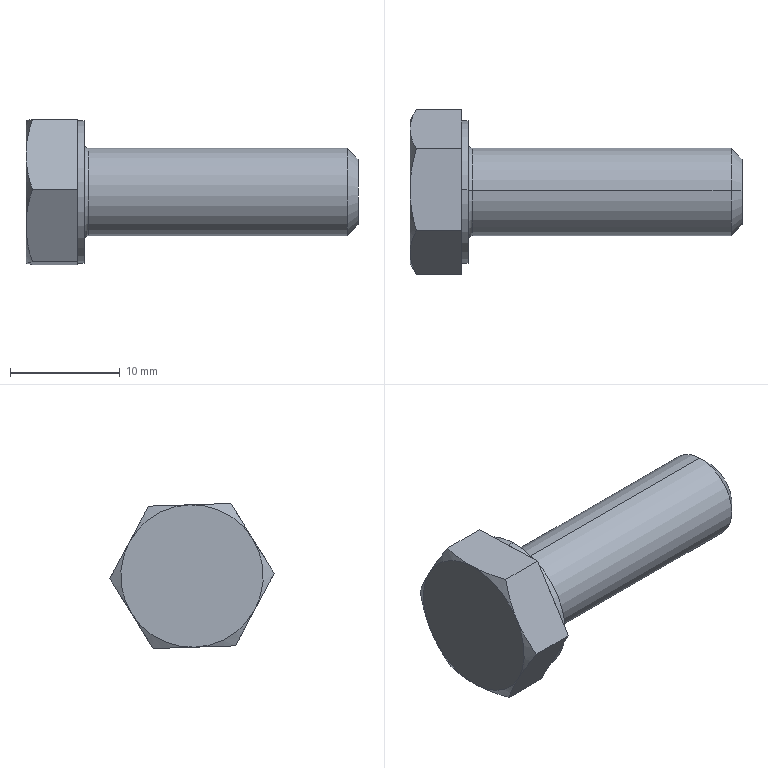Component | SolidWorks | GB_T5781-2000HexHeadBoltFullThreadC-gradeM8_25-1 | 1 solid | 29 faces | box 30.3 x 15 x 13.24 mm | volume 2011 mm3 | plane 15 | cone 8 | cylinder 4 | torus 2 | commonest cylinder face diameters 8 x2 13 x2
STEP:
#1=CARTESIAN_POINT('',(-21.77,0.005166,0.1574));
#2=VERTEX_POINT('',#1);
#3=CARTESIAN_POINT('',(-21.77,-0.005166,-0.1574));
#4=VERTEX_POINT('',#3);
#5=CARTESIAN_POINT('',(-21.77,0.,0.));
#6=DIRECTION('',(1.,0.,0.));
#7=DIRECTION('',(0.,-0.03281,-0.9995));
#8=AXIS2_PLACEMENT_3D('',#5,#6,#7);
#9=CIRCLE('',#8,0.1575);
#10=EDGE_CURVE('',#2,#4,#9,.T.);
#11=ORIENTED_EDGE('',*,*,#10,.F.);
#12=CARTESIAN_POINT('',(-21.786,0.005683,0.1731));
#13=VERTEX_POINT('',#12);
#14=CARTESIAN_POINT('',(-21.77,0.005683,0.1731));
#15=DIRECTION('',(0.,0.9995,-0.03281));
#16=DIRECTION('',(0.,0.03281,0.9995));
#17=AXIS2_PLACEMENT_3D('',#14,#15,#16);
#18=CIRCLE('',#17,0.01575);
#19=EDGE_CURVE('',#2,#13,#18,.T.);
#20=ORIENTED_EDGE('',*,*,#19,.T.);
#21=CARTESIAN_POINT('',(-21.786,-0.005683,-0.1731));
#22=VERTEX_POINT('',#21);
#23=CARTESIAN_POINT('',(-21.786,0.,0.));
#24=DIRECTION('',(-1.,0.,0.));
#25=DIRECTION('',(0.,-0.03281,-0.9995));
#26=AXIS2_PLACEMENT_3D('',#23,#24,#25);
#27=CIRCLE('',#26,0.1732);
#28=EDGE_CURVE('',#22,#13,#27,.T.);
#29=ORIENTED_EDGE('',*,*,#28,.F.);
#30=CARTESIAN_POINT('',(-21.77,-0.005683,-0.1731));
#31=DIRECTION('',(0.,-0.9995,0.03281));
#32=DIRECTION('',(0.,-0.03281,-0.9995));
#33=AXIS2_PLACEMENT_3D('',#30,#31,#32);
#34=CIRCLE('',#33,0.01575);
#35=EDGE_CURVE('',#4,#22,#34,.T.);
#36=ORIENTED_EDGE('',*,*,#35,.F.);
#37=EDGE_LOOP('',(#11,#20,#29,#36));
#38=FACE_OUTER_BOUND('',#37,.T.);
#39=CARTESIAN_POINT('',(-21.77,0.,0.));
#40=DIRECTION('',(1.,0.,0.));
#41=DIRECTION('',(0.,-0.03281,-0.9995));
#42=AXIS2_PLACEMENT_3D('',#39,#40,#41);
#43=TOROIDAL_SURFACE('',#42,0.1732,0.01575);
#44=ADVANCED_FACE('',(#38),#43,.F.);
#45=CARTESIAN_POINT('',(-20.802,-0.003875,-0.118));
#46=VERTEX_POINT('',#45);
#47=CARTESIAN_POINT('',(-20.802,0.003875,0.118));
#48=VERTEX_POINT('',#47);
#49=CARTESIAN_POINT('',(-20.802,0.,0.));
#50=DIRECTION('',(1.,0.,0.));
#51=DIRECTION('',(0.,0.03281,0.9995));
#52=AXIS2_PLACEMENT_3D('',#49,#50,#51);
#53=CIRCLE('',#52,0.1181);
#54=EDGE_CURVE('',#46,#48,#53,.T.);
#55=ORIENTED_EDGE('',*,*,#54,.F.);
#56=CARTESIAN_POINT('',(-20.841,-0.005166,-0.1574));
#57=VERTEX_POINT('',#56);
#58=CARTESIAN_POINT('',(-20.841,-0.005166,-0.1574));
#59=DIRECTION('',(-0.7071,-0.0232,-0.7067));
#60=VECTOR('',#59,39.37);
#61=LINE('',#58,#60);
#62=EDGE_CURVE('',#46,#57,#61,.T.);
#63=ORIENTED_EDGE('',*,*,#62,.T.);
#64=CARTESIAN_POINT('',(-20.841,0.005166,0.1574));
#65=VERTEX_POINT('',#64);
#66=CARTESIAN_POINT('',(-20.841,0.,0.));
#67=DIRECTION('',(-1.,0.,0.));
#68=DIRECTION('',(0.,0.03281,0.9995));
#69=AXIS2_PLACEMENT_3D('',#66,#67,#68);
#70=CIRCLE('',#69,0.1575);
#71=EDGE_CURVE('',#65,#57,#70,.T.);
#72=ORIENTED_EDGE('',*,*,#71,.F.);
#73=CARTESIAN_POINT('',(-20.841,0.005166,0.1574));
#74=DIRECTION('',(-0.7071,0.0232,0.7067));
#75=VECTOR('',#74,39.37);
#76=LINE('',#73,#75);
#77=EDGE_CURVE('',#48,#65,#76,.T.);
#78=ORIENTED_EDGE('',*,*,#77,.F.);
#79=EDGE_LOOP('',(#55,#63,#72,#78));
#80=FACE_OUTER_BOUND('',#79,.T.);
#81=CARTESIAN_POINT('',(-20.841,0.,0.));
#82=DIRECTION('',(-1.,0.,0.));
#83=DIRECTION('',(0.,0.03281,0.9995));
#84=AXIS2_PLACEMENT_3D('',#81,#82,#83);
#85=CONICAL_SURFACE('',#84,0.1575,0.7854);
#86=ADVANCED_FACE('',(#80),#85,.T.);
#87=ORIENTED_EDGE('',*,*,#71,.T.);
#88=CARTESIAN_POINT('',(-21.995,-0.005166,-0.1574));
#89=DIRECTION('',(-1.,0.,0.));
#90=VECTOR('',#89,39.37);
#91=LINE('',#88,#90);
#92=EDGE_CURVE('',#57,#4,#91,.T.);
#93=ORIENTED_EDGE('',*,*,#92,.T.);
#94=CARTESIAN_POINT('',(-21.77,0.,0.));
#95=DIRECTION('',(1.,0.,0.));
#96=DIRECTION('',(0.,-0.03281,-0.9995));
#97=AXIS2_PLACEMENT_3D('',#94,#95,#96);
#98=CIRCLE('',#97,0.1575);
#99=EDGE_CURVE('',#4,#2,#98,.T.);
#100=ORIENTED_EDGE('',*,*,#99,.T.);
#101=CARTESIAN_POINT('',(-21.995,0.005166,0.1574));
#102=DIRECTION('',(-1.,0.,0.));
#103=VECTOR('',#102,39.37);
#104=LINE('',#101,#103);
#105=EDGE_CURVE('',#65,#2,#104,.T.);
#106=ORIENTED_EDGE('',*,*,#105,.F.);
#107=EDGE_LOOP('',(#87,#93,#100,#106));
#108=FACE_OUTER_BOUND('',#107,.T.);
#109=CARTESIAN_POINT('',(-21.995,0.,0.));
#110=DIRECTION('',(-1.,0.,0.));
#111=DIRECTION('',(0.,0.03281,0.9995));
#112=AXIS2_PLACEMENT_3D('',#109,#110,#111);
#113=CYLINDRICAL_SURFACE('',#112,0.1575);
#114=ADVANCED_FACE('',(#108),#113,.T.);
#115=CARTESIAN_POINT('',(-21.786,-0.008395,-0.2558));
#116=VERTEX_POINT('',#115);
#117=CARTESIAN_POINT('',(-21.786,0.008395,0.2558));
#118=VERTEX_POINT('',#117);
#119=CARTESIAN_POINT('',(-21.786,0.,0.));
#120=DIRECTION('',(1.,0.,0.));
#121=DIRECTION('',(0.,-0.03281,-0.9995));
#122=AXIS2_PLACEMENT_3D('',#119,#120,#121);
#123=CIRCLE('',#122,0.2559);
#124=EDGE_CURVE('',#116,#118,#123,.T.);
#125=ORIENTED_EDGE('',*,*,#124,.F.);
#126=CARTESIAN_POINT('',(-21.81,-0.008395,-0.2558));
#127=VERTEX_POINT('',#126);
#128=CARTESIAN_POINT('',(-21.995,-0.008395,-0.2558));
#129=DIRECTION('',(-1.,0.,0.));
#130=VECTOR('',#129,39.37);
#131=LINE('',#128,#130);
#132=EDGE_CURVE('',#116,#127,#131,.T.);
#133=ORIENTED_EDGE('',*,*,#132,.T.);
#134=CARTESIAN_POINT('',(-21.81,0.2173,-0.1352));
#135=VERTEX_POINT('',#134);
#136=CARTESIAN_POINT('',(-21.81,0.,0.));
#137=DIRECTION('',(-1.,0.,0.));
#138=DIRECTION('',(0.,0.03281,0.9995));
#139=AXIS2_PLACEMENT_3D('',#136,#137,#138);
#140=CIRCLE('',#139,0.2559);
#141=EDGE_CURVE('',#135,#127,#140,.T.);
#142=ORIENTED_EDGE('',*,*,#141,.F.);
#143=CARTESIAN_POINT('',(-21.81,0.2257,0.1206));
#144=VERTEX_POINT('',#143);
#145=CARTESIAN_POINT('',(-21.81,0.,0.));
#146=DIRECTION('',(-1.,0.,0.));
#147=DIRECTION('',(0.,0.03281,0.9995));
#148=AXIS2_PLACEMENT_3D('',#145,#146,#147);
#149=CIRCLE('',#148,0.2559);
#150=EDGE_CURVE('',#144,#135,#149,.T.);
#151=ORIENTED_EDGE('',*,*,#150,.F.);
#152=CARTESIAN_POINT('',(-21.81,0.008395,0.2558));
#153=VERTEX_POINT('',#152);
#154=CARTESIAN_POINT('',(-21.81,0.,0.));
#155=DIRECTION('',(-1.,0.,0.));
#156=DIRECTION('',(0.,0.03281,0.9995));
#157=AXIS2_PLACEMENT_3D('',#154,#155,#156);
#158=CIRCLE('',#157,0.2559);
#159=EDGE_CURVE('',#153,#144,#158,.T.);
#160=ORIENTED_EDGE('',*,*,#159,.F.);
#161=CARTESIAN_POINT('',(-21.995,0.008395,0.2558));
#162=DIRECTION('',(-1.,0.,0.));
#163=VECTOR('',#162,39.37);
#164=LINE('',#161,#163);
#165=EDGE_CURVE('',#118,#153,#164,.T.);
#166=ORIENTED_EDGE('',*,*,#165,.F.);
#167=EDGE_LOOP('',(#125,#133,#142,#151,#160,#166));
#168=FACE_OUTER_BOUND('',#167,.T.);
#169=CARTESIAN_POINT('',(-21.995,0.,0.));
#170=DIRECTION('',(-1.,0.,0.));
#171=DIRECTION('',(0.,0.03281,0.9995));
#172=AXIS2_PLACEMENT_3D('',#169,#170,#171);
#173=CYLINDRICAL_SURFACE('',#172,0.2559);
#174=ADVANCED_FACE('',(#168),#173,.T.);
#175=CARTESIAN_POINT('',(-21.81,0.1393,-0.2606));
#176=VERTEX_POINT('',#175);
#177=CARTESIAN_POINT('',(-21.81,0.1393,-0.2606));
#178=DIRECTION('',(0.,0.5281,0.8492));
#179=VECTOR('',#178,39.37);
#180=LINE('',#177,#179);
#181=EDGE_CURVE('',#176,#135,#180,.T.);
#182=ORIENTED_EDGE('',*,*,#181,.F.);
#183=CARTESIAN_POINT('',(-21.972,0.1393,-0.2606));
#184=VERTEX_POINT('',#183);
#185=CARTESIAN_POINT('',(-21.786,0.1393,-0.2606));
#186=DIRECTION('',(-1.,0.,0.));
#187=VECTOR('',#186,39.37);
#188=LINE('',#185,#187);
#189=EDGE_CURVE('',#176,#184,#188,.T.);
#190=ORIENTED_EDGE('',*,*,#189,.T.);
#191=CARTESIAN_POINT('',(-21.995,0.2173,-0.1352));
#192=VERTEX_POINT('',#191);
#193=CARTESIAN_POINT('',(-21.995,0.2173,-0.1352));
#194=CARTESIAN_POINT('',(-21.995,0.2107,-0.1458));
#195=CARTESIAN_POINT('',(-21.994,0.204,-0.1565));
#196=CARTESIAN_POINT('',(-21.992,0.1909,-0.1777));
#197=CARTESIAN_POINT('',(-21.99,0.1843,-0.1882));
#198=CARTESIAN_POINT('',(-21.985,0.1648,-0.2195));
#199=CARTESIAN_POINT('',(-21.979,0.152,-0.2401));
#200=CARTESIAN_POINT('',(-21.972,0.1393,-0.2606));
#201=B_SPLINE_CURVE_WITH_KNOTS('',3,(#193,#194,#195,#196,#197,#198,#199,#200),.UNSPECIFIED.,.F.,.F.,(4,2,2,4),(0.003797,0.004743,0.005689,0.00758),.UNSPECIFIED.);
#202=EDGE_CURVE('',#192,#184,#201,.T.);
#203=ORIENTED_EDGE('',*,*,#202,.F.);
#204=CARTESIAN_POINT('',(-21.972,0.2953,-0.009694));
#205=VERTEX_POINT('',#204);
#206=CARTESIAN_POINT('',(-21.972,0.2953,-0.009694));
#207=CARTESIAN_POINT('',(-21.979,0.2826,-0.03022));
#208=CARTESIAN_POINT('',(-21.985,0.2697,-0.05089));
#209=CARTESIAN_POINT('',(-21.992,0.2437,-0.09267));
#210=CARTESIAN_POINT('',(-21.995,0.2306,-0.1138));
#211=CARTESIAN_POINT('',(-21.995,0.2173,-0.1352));
#212=B_SPLINE_CURVE_WITH_KNOTS('',3,(#206,#207,#208,#209,#210,#211),.UNSPECIFIED.,.F.,.F.,(4,2,4),(0.00000024,0.001899,0.003797),.UNSPECIFIED.);
#213=EDGE_CURVE('',#205,#192,#212,.T.);
#214=ORIENTED_EDGE('',*,*,#213,.F.);
#215=CARTESIAN_POINT('',(-21.81,0.2953,-0.009694));
#216=VERTEX_POINT('',#215);
#217=CARTESIAN_POINT('',(-21.786,0.2953,-0.009694));
#218=DIRECTION('',(-1.,0.,0.));
#219=VECTOR('',#218,39.37);
#220=LINE('',#217,#219);
#221=EDGE_CURVE('',#216,#205,#220,.T.);
#222=ORIENTED_EDGE('',*,*,#221,.F.);
#223=CARTESIAN_POINT('',(-21.81,0.1393,-0.2606));
#224=DIRECTION('',(0.,0.5281,0.8492));
#225=VECTOR('',#224,39.37);
#226=LINE('',#223,#225);
#227=EDGE_CURVE('',#135,#216,#226,.T.);
#228=ORIENTED_EDGE('',*,*,#227,.F.);
#229=EDGE_LOOP('',(#182,#190,#203,#214,#222,#228));
#230=FACE_OUTER_BOUND('',#229,.T.);
#231=CARTESIAN_POINT('',(-21.786,0.1393,-0.2606));
#232=DIRECTION('',(0.,-0.8492,0.5281));
#233=DIRECTION('',(0.,-0.5281,-0.8492));
#234=AXIS2_PLACEMENT_3D('',#231,#232,#233);
#235=PLANE('',#234);
#236=ADVANCED_FACE('',(#230),#235,.F.);
#237=CARTESIAN_POINT('',(-21.81,0.2953,-0.009694));
#238=DIRECTION('',(0.,-0.4713,0.882));
#239=VECTOR('',#238,39.37);
#240=LINE('',#237,#239);
#241=EDGE_CURVE('',#216,#144,#240,.T.);
#242=ORIENTED_EDGE('',*,*,#241,.F.);
#243=ORIENTED_EDGE('',*,*,#221,.T.);
#244=CARTESIAN_POINT('',(-21.995,0.2257,0.1206));
#245=VERTEX_POINT('',#244);
#246=CARTESIAN_POINT('',(-21.995,0.2257,0.1206));
#247=CARTESIAN_POINT('',(-21.995,0.2316,0.1096));
#248=CARTESIAN_POINT('',(-21.994,0.2375,0.09845));
#249=CARTESIAN_POINT('',(-21.992,0.2493,0.07647));
#250=CARTESIAN_POINT('',(-21.99,0.2551,0.06556));
#251=CARTESIAN_POINT('',(-21.985,0.2725,0.03301));
#252=CARTESIAN_POINT('',(-21.979,0.284,0.01157));
#253=CARTESIAN_POINT('',(-21.972,0.2953,-0.009694));
#254=B_SPLINE_CURVE_WITH_KNOTS('',3,(#246,#247,#248,#249,#250,#251,#252,#253),.UNSPECIFIED.,.F.,.F.,(4,2,2,4),(0.003797,0.004743,0.005689,0.00758),.UNSPECIFIED.);
#255=EDGE_CURVE('',#245,#205,#254,.T.);
#256=ORIENTED_EDGE('',*,*,#255,.F.);
#257=CARTESIAN_POINT('',(-21.972,0.1561,0.2509));
#258=VERTEX_POINT('',#257);
#259=CARTESIAN_POINT('',(-21.972,0.1561,0.2509));
#260=CARTESIAN_POINT('',(-21.979,0.1675,0.2296));
#261=CARTESIAN_POINT('',(-21.985,0.1789,0.2081));
#262=CARTESIAN_POINT('',(-21.992,0.2021,0.1647));
#263=CARTESIAN_POINT('',(-21.995,0.2138,0.1428));
#264=CARTESIAN_POINT('',(-21.995,0.2257,0.1206));
#265=B_SPLINE_CURVE_WITH_KNOTS('',3,(#259,#260,#261,#262,#263,#264),.UNSPECIFIED.,.F.,.F.,(4,2,4),(0.00000024,0.001899,0.003797),.UNSPECIFIED.);
#266=EDGE_CURVE('',#258,#245,#265,.T.);
#267=ORIENTED_EDGE('',*,*,#266,.F.);
#268=CARTESIAN_POINT('',(-21.81,0.1561,0.2509));
#269=VERTEX_POINT('',#268);
#270=CARTESIAN_POINT('',(-21.786,0.1561,0.2509));
#271=DIRECTION('',(-1.,0.,0.));
#272=VECTOR('',#271,39.37);
#273=LINE('',#270,#272);
#274=EDGE_CURVE('',#269,#258,#273,.T.);
#275=ORIENTED_EDGE('',*,*,#274,.F.);
#276=CARTESIAN_POINT('',(-21.81,0.2953,-0.009694));
#277=DIRECTION('',(0.,-0.4713,0.882));
#278=VECTOR('',#277,39.37);
#279=LINE('',#276,#278);
#280=EDGE_CURVE('',#144,#269,#279,.T.);
#281=ORIENTED_EDGE('',*,*,#280,.F.);
#282=EDGE_LOOP('',(#242,#243,#256,#267,#275,#281));
#283=FACE_OUTER_BOUND('',#282,.T.);
#284=CARTESIAN_POINT('',(-21.786,0.2953,-0.009694));
#285=DIRECTION('',(0.,-0.882,-0.4713));
#286=DIRECTION('',(0.,0.4713,-0.882));
#287=AXIS2_PLACEMENT_3D('',#284,#285,#286);
#288=PLANE('',#287);
#289=ADVANCED_FACE('',(#283),#288,.F.);
#290=CARTESIAN_POINT('',(-21.81,0.1561,0.2509));
#291=DIRECTION('',(0.,-0.9995,0.03281));
#292=VECTOR('',#291,39.37);
#293=LINE('',#290,#292);
#294=EDGE_CURVE('',#269,#153,#293,.T.);
#295=ORIENTED_EDGE('',*,*,#294,.F.);
#296=ORIENTED_EDGE('',*,*,#274,.T.);
#297=CARTESIAN_POINT('',(-21.995,0.008395,0.2558));
#298=VERTEX_POINT('',#297);
#299=CARTESIAN_POINT('',(-21.995,0.008395,0.2558));
#300=CARTESIAN_POINT('',(-21.995,0.03339,0.2549));
#301=CARTESIAN_POINT('',(-21.992,0.0587,0.2541));
#302=CARTESIAN_POINT('',(-21.984,0.108,0.2525));
#303=CARTESIAN_POINT('',(-21.979,0.1322,0.2517));
#304=CARTESIAN_POINT('',(-21.972,0.1561,0.2509));
#305=B_SPLINE_CURVE_WITH_KNOTS('',3,(#299,#300,#301,#302,#303,#304),.UNSPECIFIED.,.F.,.F.,(4,2,4),(0.01067,0.01257,0.01447),.UNSPECIFIED.);
#306=EDGE_CURVE('',#298,#258,#305,.T.);
#307=ORIENTED_EDGE('',*,*,#306,.F.);
#308=CARTESIAN_POINT('',(-21.972,-0.1393,0.2606));
#309=VERTEX_POINT('',#308);
#310=CARTESIAN_POINT('',(-21.972,-0.1393,0.2606));
#311=CARTESIAN_POINT('',(-21.979,-0.1152,0.2598));
#312=CARTESIAN_POINT('',(-21.985,-0.09065,0.259));
#313=CARTESIAN_POINT('',(-21.993,-0.04137,0.2574));
#314=CARTESIAN_POINT('',(-21.995,-0.01658,0.2566));
#315=CARTESIAN_POINT('',(-21.995,0.008395,0.2558));
#316=B_SPLINE_CURVE_WITH_KNOTS('',3,(#310,#311,#312,#313,#314,#315),.UNSPECIFIED.,.F.,.F.,(4,2,4),(0.006874,0.008773,0.01067),.UNSPECIFIED.);
#317=EDGE_CURVE('',#309,#298,#316,.T.);
#318=ORIENTED_EDGE('',*,*,#317,.F.);
#319=CARTESIAN_POINT('',(-21.81,-0.1393,0.2606));
#320=VERTEX_POINT('',#319);
#321=CARTESIAN_POINT('',(-21.786,-0.1393,0.2606));
#322=DIRECTION('',(-1.,0.,0.));
#323=VECTOR('',#322,39.37);
#324=LINE('',#321,#323);
#325=EDGE_CURVE('',#320,#309,#324,.T.);
#326=ORIENTED_EDGE('',*,*,#325,.F.);
#327=CARTESIAN_POINT('',(-21.81,0.1561,0.2509));
#328=DIRECTION('',(0.,-0.9995,0.03281));
#329=VECTOR('',#328,39.37);
#330=LINE('',#327,#329);
#331=EDGE_CURVE('',#153,#320,#330,.T.);
#332=ORIENTED_EDGE('',*,*,#331,.F.);
#333=EDGE_LOOP('',(#295,#296,#307,#318,#326,#332));
#334=FACE_OUTER_BOUND('',#333,.T.);
#335=CARTESIAN_POINT('',(-21.786,0.1561,0.2509));
#336=DIRECTION('',(0.,-0.03281,-0.9995));
#337=DIRECTION('',(0.,0.9995,-0.03281));
#338=AXIS2_PLACEMENT_3D('',#335,#336,#337);
#339=PLANE('',#338);
#340=ADVANCED_FACE('',(#334),#339,.F.);
#341=CARTESIAN_POINT('',(-21.81,-0.2173,0.1352));
#342=VERTEX_POINT('',#341);
#343=CARTESIAN_POINT('',(-21.81,-0.2953,0.009694));
#344=DIRECTION('',(0.,-0.5281,-0.8492));
#345=VECTOR('',#344,39.37);
#346=LINE('',#343,#345);
#347=EDGE_CURVE('',#320,#342,#346,.T.);
#348=ORIENTED_EDGE('',*,*,#347,.F.);
#349=ORIENTED_EDGE('',*,*,#325,.T.);
#350=CARTESIAN_POINT('',(-21.995,-0.2173,0.1352));
#351=VERTEX_POINT('',#350);
#352=CARTESIAN_POINT('',(-21.995,-0.2173,0.1352));
#353=CARTESIAN_POINT('',(-21.995,-0.2107,0.1458));
#354=CARTESIAN_POINT('',(-21.994,-0.204,0.1565));
#355=CARTESIAN_POINT('',(-21.992,-0.1909,0.1777));
#356=CARTESIAN_POINT('',(-21.99,-0.1843,0.1882));
#357=CARTESIAN_POINT('',(-21.985,-0.1648,0.2195));
#358=CARTESIAN_POINT('',(-21.979,-0.152,0.2401));
#359=CARTESIAN_POINT('',(-21.972,-0.1393,0.2606));
#360=B_SPLINE_CURVE_WITH_KNOTS('',3,(#352,#353,#354,#355,#356,#357,#358,#359),.UNSPECIFIED.,.F.,.F.,(4,2,2,4),(0.003797,0.004743,0.005689,0.00758),.UNSPECIFIED.);
#361=EDGE_CURVE('',#351,#309,#360,.T.);
#362=ORIENTED_EDGE('',*,*,#361,.F.);
#363=CARTESIAN_POINT('',(-21.972,-0.2953,0.009694));
#364=VERTEX_POINT('',#363);
#365=CARTESIAN_POINT('',(-21.972,-0.2953,0.009694));
#366=CARTESIAN_POINT('',(-21.979,-0.2826,0.03022));
#367=CARTESIAN_POINT('',(-21.985,-0.2697,0.05089));
#368=CARTESIAN_POINT('',(-21.992,-0.2437,0.09267));
#369=CARTESIAN_POINT('',(-21.995,-0.2306,0.1138));
#370=CARTESIAN_POINT('',(-21.995,-0.2173,0.1352));
#371=B_SPLINE_CURVE_WITH_KNOTS('',3,(#365,#366,#367,#368,#369,#370),.UNSPECIFIED.,.F.,.F.,(4,2,4),(0.00000024,0.001899,0.003797),.UNSPECIFIED.);
#372=EDGE_CURVE('',#364,#351,#371,.T.);
#373=ORIENTED_EDGE('',*,*,#372,.F.);
#374=CARTESIAN_POINT('',(-21.81,-0.2953,0.009694));
#375=VERTEX_POINT('',#374);
#376=CARTESIAN_POINT('',(-21.786,-0.2953,0.009694));
#377=DIRECTION('',(-1.,0.,0.));
#378=VECTOR('',#377,39.37);
#379=LINE('',#376,#378);
#380=EDGE_CURVE('',#375,#364,#379,.T.);
#381=ORIENTED_EDGE('',*,*,#380,.F.);
#382=CARTESIAN_POINT('',(-21.81,-0.2953,0.009694));
#383=DIRECTION('',(0.,-0.5281,-0.8492));
#384=VECTOR('',#383,39.37);
#385=LINE('',#382,#384);
#386=EDGE_CURVE('',#342,#375,#385,.T.);
#387=ORIENTED_EDGE('',*,*,#386,.F.);
#388=EDGE_LOOP('',(#348,#349,#362,#373,#381,#387));
#389=FACE_OUTER_BOUND('',#388,.T.);
#390=CARTESIAN_POINT('',(-21.786,-0.2953,0.009694));
#391=DIRECTION('',(0.,0.8492,-0.5281));
#392=DIRECTION('',(0.,0.5281,0.8492));
#393=AXIS2_PLACEMENT_3D('',#390,#391,#392);
#394=PLANE('',#393);
#395=ADVANCED_FACE('',(#389),#394,.F.);
#396=CARTESIAN_POINT('',(-21.81,-0.2257,-0.1206));
#397=VERTEX_POINT('',#396);
#398=CARTESIAN_POINT('',(-21.81,-0.1561,-0.2509));
#399=DIRECTION('',(0.,0.4713,-0.882));
#400=VECTOR('',#399,39.37);
#401=LINE('',#398,#400);
#402=EDGE_CURVE('',#375,#397,#401,.T.);
#403=ORIENTED_EDGE('',*,*,#402,.F.);
#404=ORIENTED_EDGE('',*,*,#380,.T.);
#405=CARTESIAN_POINT('',(-21.995,-0.2257,-0.1206));
#406=VERTEX_POINT('',#405);
#407=CARTESIAN_POINT('',(-21.995,-0.2257,-0.1206));
#408=CARTESIAN_POINT('',(-21.995,-0.2316,-0.1096));
#409=CARTESIAN_POINT('',(-21.994,-0.2375,-0.09845));
#410=CARTESIAN_POINT('',(-21.992,-0.2493,-0.07647));
#411=CARTESIAN_POINT('',(-21.99,-0.2551,-0.06556));
#412=CARTESIAN_POINT('',(-21.985,-0.2725,-0.03301));
#413=CARTESIAN_POINT('',(-21.979,-0.284,-0.01157));
#414=CARTESIAN_POINT('',(-21.972,-0.2953,0.009694));
#415=B_SPLINE_CURVE_WITH_KNOTS('',3,(#407,#408,#409,#410,#411,#412,#413,#414),.UNSPECIFIED.,.F.,.F.,(4,2,2,4),(0.003797,0.004743,0.005689,0.00758),.UNSPECIFIED.);
#416=EDGE_CURVE('',#406,#364,#415,.T.);
#417=ORIENTED_EDGE('',*,*,#416,.F.);
#418=CARTESIAN_POINT('',(-21.972,-0.1561,-0.2509));
#419=VERTEX_POINT('',#418);
#420=CARTESIAN_POINT('',(-21.972,-0.1561,-0.2509));
#421=CARTESIAN_POINT('',(-21.979,-0.1675,-0.2296));
#422=CARTESIAN_POINT('',(-21.985,-0.1789,-0.2081));
#423=CARTESIAN_POINT('',(-21.992,-0.2021,-0.1647));
#424=CARTESIAN_POINT('',(-21.995,-0.2138,-0.1428));
#425=CARTESIAN_POINT('',(-21.995,-0.2257,-0.1206));
#426=B_SPLINE_CURVE_WITH_KNOTS('',3,(#420,#421,#422,#423,#424,#425),.UNSPECIFIED.,.F.,.F.,(4,2,4),(0.00000024,0.001899,0.003797),.UNSPECIFIED.);
#427=EDGE_CURVE('',#419,#406,#426,.T.);
#428=ORIENTED_EDGE('',*,*,#427,.F.);
#429=CARTESIAN_POINT('',(-21.81,-0.1561,-0.2509));
#430=VERTEX_POINT('',#429);
#431=CARTESIAN_POINT('',(-21.786,-0.1561,-0.2509));
#432=DIRECTION('',(-1.,0.,0.));
#433=VECTOR('',#432,39.37);
#434=LINE('',#431,#433);
#435=EDGE_CURVE('',#430,#419,#434,.T.);
#436=ORIENTED_EDGE('',*,*,#435,.F.);
#437=CARTESIAN_POINT('',(-21.81,-0.1561,-0.2509));
#438=DIRECTION('',(0.,0.4713,-0.882));
#439=VECTOR('',#438,39.37);
#440=LINE('',#437,#439);
#441=EDGE_CURVE('',#397,#430,#440,.T.);
#442=ORIENTED_EDGE('',*,*,#441,.F.);
#443=EDGE_LOOP('',(#403,#404,#417,#428,#436,#442));
#444=FACE_OUTER_BOUND('',#443,.T.);
#445=CARTESIAN_POINT('',(-21.786,-0.1561,-0.2509));
#446=DIRECTION('',(0.,0.882,0.4713));
#447=DIRECTION('',(0.,-0.4713,0.882));
#448=AXIS2_PLACEMENT_3D('',#445,#446,#447);
#449=PLANE('',#448);
#450=ADVANCED_FACE('',(#444),#449,.F.);
#451=CARTESIAN_POINT('',(-21.81,0.1393,-0.2606));
#452=DIRECTION('',(0.,0.9995,-0.03281));
#453=VECTOR('',#452,39.37);
#454=LINE('',#451,#453);
#455=EDGE_CURVE('',#430,#127,#454,.T.);
#456=ORIENTED_EDGE('',*,*,#455,.F.);
#457=ORIENTED_EDGE('',*,*,#435,.T.);
#458=CARTESIAN_POINT('',(-21.995,-0.008395,-0.2558));
#459=VERTEX_POINT('',#458);
#460=CARTESIAN_POINT('',(-21.995,-0.008395,-0.2558));
#461=CARTESIAN_POINT('',(-21.995,-0.03337,-0.2549));
#462=CARTESIAN_POINT('',(-21.993,-0.05816,-0.2541));
#463=CARTESIAN_POINT('',(-21.985,-0.1074,-0.2525));
#464=CARTESIAN_POINT('',(-21.979,-0.132,-0.2517));
#465=CARTESIAN_POINT('',(-21.972,-0.1561,-0.2509));
#466=B_SPLINE_CURVE_WITH_KNOTS('',3,(#460,#461,#462,#463,#464,#465),.UNSPECIFIED.,.F.,.F.,(4,2,4),(0.02294,0.02484,0.02674),.UNSPECIFIED.);
#467=EDGE_CURVE('',#459,#419,#466,.T.);
#468=ORIENTED_EDGE('',*,*,#467,.F.);
#469=CARTESIAN_POINT('',(-21.972,0.1393,-0.2606));
#470=CARTESIAN_POINT('',(-21.979,0.1154,-0.2598));
#471=CARTESIAN_POINT('',(-21.984,0.0912,-0.259));
#472=CARTESIAN_POINT('',(-21.992,0.04191,-0.2574));
#473=CARTESIAN_POINT('',(-21.995,0.0166,-0.2566));
#474=CARTESIAN_POINT('',(-21.995,-0.008395,-0.2558));
#475=B_SPLINE_CURVE_WITH_KNOTS('',3,(#469,#470,#471,#472,#473,#474),.UNSPECIFIED.,.F.,.F.,(4,2,4),(0.01914,0.02104,0.02294),.UNSPECIFIED.);
#476=EDGE_CURVE('',#184,#459,#475,.T.);
#477=ORIENTED_EDGE('',*,*,#476,.F.);
#478=ORIENTED_EDGE('',*,*,#189,.F.);
#479=CARTESIAN_POINT('',(-21.81,0.1393,-0.2606));
#480=DIRECTION('',(0.,0.9995,-0.03281));
#481=VECTOR('',#480,39.37);
#482=LINE('',#479,#481);
#483=EDGE_CURVE('',#127,#176,#482,.T.);
#484=ORIENTED_EDGE('',*,*,#483,.F.);
#485=EDGE_LOOP('',(#456,#457,#468,#477,#478,#484));
#486=FACE_OUTER_BOUND('',#485,.T.);
#487=CARTESIAN_POINT('',(-21.786,0.1393,-0.2606));
#488=DIRECTION('',(0.,0.03281,0.9995));
#489=DIRECTION('',(0.,-0.9995,0.03281));
#490=AXIS2_PLACEMENT_3D('',#487,#488,#489);
#491=PLANE('',#490);
#492=ADVANCED_FACE('',(#486),#491,.F.);
#493=ORIENTED_EDGE('',*,*,#427,.T.);
#494=CARTESIAN_POINT('',(-21.995,0.,0.));
#495=DIRECTION('',(1.,0.,0.));
#496=DIRECTION('',(0.,-0.03281,-0.9995));
#497=AXIS2_PLACEMENT_3D('',#494,#495,#496);
#498=CIRCLE('',#497,0.2559);
#499=EDGE_CURVE('',#406,#459,#498,.T.);
#500=ORIENTED_EDGE('',*,*,#499,.T.);
#501=ORIENTED_EDGE('',*,*,#467,.T.);
#502=EDGE_LOOP('',(#493,#500,#501));
#503=FACE_OUTER_BOUND('',#502,.T.);
#504=CARTESIAN_POINT('',(-21.995,0.,0.));
#505=DIRECTION('',(1.,0.,0.));
#506=DIRECTION('',(0.,-0.03281,-0.9995));
#507=AXIS2_PLACEMENT_3D('',#504,#505,#506);
#508=CONICAL_SURFACE('',#507,0.2559,1.047);
#509=ADVANCED_FACE('',(#503),#508,.T.);
#510=ORIENTED_EDGE('',*,*,#372,.T.);
#511=CARTESIAN_POINT('',(-21.995,0.,0.));
#512=DIRECTION('',(1.,0.,0.));
#513=DIRECTION('',(0.,-0.03281,-0.9995));
#514=AXIS2_PLACEMENT_3D('',#511,#512,#513);
#515=CIRCLE('',#514,0.2559);
#516=EDGE_CURVE('',#351,#406,#515,.T.);
#517=ORIENTED_EDGE('',*,*,#516,.T.);
#518=ORIENTED_EDGE('',*,*,#416,.T.);
#519=EDGE_LOOP('',(#510,#517,#518));
#520=FACE_OUTER_BOUND('',#519,.T.);
#521=CARTESIAN_POINT('',(-21.995,0.,0.));
#522=DIRECTION('',(1.,0.,0.));
#523=DIRECTION('',(0.,-0.03281,-0.9995));
#524=AXIS2_PLACEMENT_3D('',#521,#522,#523);
#525=CONICAL_SURFACE('',#524,0.2559,1.047);
#526=ADVANCED_FACE('',(#520),#525,.T.);
#527=ORIENTED_EDGE('',*,*,#317,.T.);
#528=CARTESIAN_POINT('',(-21.995,0.,0.));
#529=DIRECTION('',(1.,0.,0.));
#530=DIRECTION('',(0.,-0.03281,-0.9995));
#531=AXIS2_PLACEMENT_3D('',#528,#529,#530);
#532=CIRCLE('',#531,0.2559);
#533=EDGE_CURVE('',#298,#351,#532,.T.);
#534=ORIENTED_EDGE('',*,*,#533,.T.);
#535=ORIENTED_EDGE('',*,*,#361,.T.);
#536=EDGE_LOOP('',(#527,#534,#535));
#537=FACE_OUTER_BOUND('',#536,.T.);
#538=CARTESIAN_POINT('',(-21.995,0.,0.));
#539=DIRECTION('',(1.,0.,0.));
#540=DIRECTION('',(0.,-0.03281,-0.9995));
#541=AXIS2_PLACEMENT_3D('',#538,#539,#540);
#542=CONICAL_SURFACE('',#541,0.2559,1.047);
#543=ADVANCED_FACE('',(#537),#542,.T.);
#544=ORIENTED_EDGE('',*,*,#306,.T.);
#545=ORIENTED_EDGE('',*,*,#266,.T.);
#546=CARTESIAN_POINT('',(-21.995,0.,0.));
#547=DIRECTION('',(-1.,0.,0.));
#548=DIRECTION('',(0.,0.03281,0.9995));
#549=AXIS2_PLACEMENT_3D('',#546,#547,#548);
#550=CIRCLE('',#549,0.2559);
#551=EDGE_CURVE('',#298,#245,#550,.T.);
#552=ORIENTED_EDGE('',*,*,#551,.F.);
#553=EDGE_LOOP('',(#544,#545,#552));
#554=FACE_OUTER_BOUND('',#553,.T.);
#555=CARTESIAN_POINT('',(-21.995,0.,0.));
#556=DIRECTION('',(1.,0.,0.));
#557=DIRECTION('',(0.,-0.03281,-0.9995));
#558=AXIS2_PLACEMENT_3D('',#555,#556,#557);
#559=CONICAL_SURFACE('',#558,0.2559,1.047);
#560=ADVANCED_FACE('',(#554),#559,.T.);
#561=ORIENTED_EDGE('',*,*,#255,.T.);
#562=ORIENTED_EDGE('',*,*,#213,.T.);
#563=CARTESIAN_POINT('',(-21.995,0.,0.));
#564=DIRECTION('',(1.,0.,0.));
#565=DIRECTION('',(0.,-0.03281,-0.9995));
#566=AXIS2_PLACEMENT_3D('',#563,#564,#565);
#567=CIRCLE('',#566,0.2559);
#568=EDGE_CURVE('',#192,#245,#567,.T.);
#569=ORIENTED_EDGE('',*,*,#568,.T.);
#570=EDGE_LOOP('',(#561,#562,#569));
#571=FACE_OUTER_BOUND('',#570,.T.);
#572=CARTESIAN_POINT('',(-21.995,0.,0.));
#573=DIRECTION('',(1.,0.,0.));
#574=DIRECTION('',(0.,-0.03281,-0.9995));
#575=AXIS2_PLACEMENT_3D('',#572,#573,#574);
#576=CONICAL_SURFACE('',#575,0.2559,1.047);
#577=ADVANCED_FACE('',(#571),#576,.T.);
#578=ORIENTED_EDGE('',*,*,#202,.T.);
#579=ORIENTED_EDGE('',*,*,#476,.T.);
#580=CARTESIAN_POINT('',(-21.995,0.,0.));
#581=DIRECTION('',(1.,0.,0.));
#582=DIRECTION('',(0.,-0.03281,-0.9995));
#583=AXIS2_PLACEMENT_3D('',#580,#581,#582);
#584=CIRCLE('',#583,0.2559);
#585=EDGE_CURVE('',#459,#192,#584,.T.);
#586=ORIENTED_EDGE('',*,*,#585,.T.);
#587=EDGE_LOOP('',(#578,#579,#586));
#588=FACE_OUTER_BOUND('',#587,.T.);
#589=CARTESIAN_POINT('',(-21.995,0.,0.));
#590=DIRECTION('',(1.,0.,0.));
#591=DIRECTION('',(0.,-0.03281,-0.9995));
#592=AXIS2_PLACEMENT_3D('',#589,#590,#591);
#593=CONICAL_SURFACE('',#592,0.2559,1.047);
#594=ADVANCED_FACE('',(#588),#593,.T.);
#595=ORIENTED_EDGE('',*,*,#585,.F.);
#596=ORIENTED_EDGE('',*,*,#499,.F.);
#597=ORIENTED_EDGE('',*,*,#516,.F.);
#598=ORIENTED_EDGE('',*,*,#533,.F.);
#599=ORIENTED_EDGE('',*,*,#551,.T.);
#600=ORIENTED_EDGE('',*,*,#568,.F.);
#601=EDGE_LOOP('',(#595,#596,#597,#598,#599,#600));
#602=FACE_OUTER_BOUND('',#601,.T.);
#603=CARTESIAN_POINT('',(-21.995,0.2953,-0.009694));
#604=DIRECTION('',(1.,0.,0.));
#605=DIRECTION('',(0.,-0.03281,-0.9995));
#606=AXIS2_PLACEMENT_3D('',#603,#604,#605);
#607=PLANE('',#606);
#608=ADVANCED_FACE('',(#602),#607,.F.);
#609=ORIENTED_EDGE('',*,*,#181,.T.);
#610=ORIENTED_EDGE('',*,*,#141,.T.);
#611=ORIENTED_EDGE('',*,*,#483,.T.);
#612=EDGE_LOOP('',(#609,#610,#611));
#613=FACE_OUTER_BOUND('',#612,.T.);
#614=CARTESIAN_POINT('',(-21.81,0.2558,-0.008395));
#615=DIRECTION('',(1.,0.,0.));
#616=DIRECTION('',(0.,-0.03281,-0.9995));
#617=AXIS2_PLACEMENT_3D('',#614,#615,#616);
#618=PLANE('',#617);
#619=ADVANCED_FACE('',(#613),#618,.T.);
#620=ORIENTED_EDGE('',*,*,#227,.T.);
#621=ORIENTED_EDGE('',*,*,#241,.T.);
#622=ORIENTED_EDGE('',*,*,#150,.T.);
#623=EDGE_LOOP('',(#620,#621,#622));
#624=FACE_OUTER_BOUND('',#623,.T.);
#625=CARTESIAN_POINT('',(-21.81,0.2558,-0.008395));
#626=DIRECTION('',(1.,0.,0.));
#627=DIRECTION('',(0.,-0.03281,-0.9995));
#628=AXIS2_PLACEMENT_3D('',#625,#626,#627);
#629=PLANE('',#628);
#630=ADVANCED_FACE('',(#624),#629,.T.);
#631=ORIENTED_EDGE('',*,*,#280,.T.);
#632=ORIENTED_EDGE('',*,*,#294,.T.);
#633=ORIENTED_EDGE('',*,*,#159,.T.);
#634=EDGE_LOOP('',(#631,#632,#633));
#635=FACE_OUTER_BOUND('',#634,.T.);
#636=CARTESIAN_POINT('',(-21.81,0.2558,-0.008395));
#637=DIRECTION('',(1.,0.,0.));
#638=DIRECTION('',(0.,-0.03281,-0.9995));
#639=AXIS2_PLACEMENT_3D('',#636,#637,#638);
#640=PLANE('',#639);
#641=ADVANCED_FACE('',(#635),#640,.T.);
#642=ORIENTED_EDGE('',*,*,#331,.T.);
#643=ORIENTED_EDGE('',*,*,#347,.T.);
#644=CARTESIAN_POINT('',(-21.81,0.,0.));
#645=DIRECTION('',(-1.,0.,0.));
#646=DIRECTION('',(0.,0.03281,0.9995));
#647=AXIS2_PLACEMENT_3D('',#644,#645,#646);
#648=CIRCLE('',#647,0.2559);
#649=EDGE_CURVE('',#342,#153,#648,.T.);
#650=ORIENTED_EDGE('',*,*,#649,.T.);
#651=EDGE_LOOP('',(#642,#643,#650));
#652=FACE_OUTER_BOUND('',#651,.T.);
#653=CARTESIAN_POINT('',(-21.81,0.2558,-0.008395));
#654=DIRECTION('',(1.,0.,0.));
#655=DIRECTION('',(0.,-0.03281,-0.9995));
#656=AXIS2_PLACEMENT_3D('',#653,#654,#655);
#657=PLANE('',#656);
#658=ADVANCED_FACE('',(#652),#657,.T.);
#659=ORIENTED_EDGE('',*,*,#386,.T.);
#660=ORIENTED_EDGE('',*,*,#402,.T.);
#661=CARTESIAN_POINT('',(-21.81,0.,0.));
#662=DIRECTION('',(-1.,0.,0.));
#663=DIRECTION('',(0.,0.03281,0.9995));
#664=AXIS2_PLACEMENT_3D('',#661,#662,#663);
#665=CIRCLE('',#664,0.2559);
#666=EDGE_CURVE('',#397,#342,#665,.T.);
#667=ORIENTED_EDGE('',*,*,#666,.T.);
#668=EDGE_LOOP('',(#659,#660,#667));
#669=FACE_OUTER_BOUND('',#668,.T.);
#670=CARTESIAN_POINT('',(-21.81,0.2558,-0.008395));
#671=DIRECTION('',(1.,0.,0.));
#672=DIRECTION('',(0.,-0.03281,-0.9995));
#673=AXIS2_PLACEMENT_3D('',#670,#671,#672);
#674=PLANE('',#673);
#675=ADVANCED_FACE('',(#669),#674,.T.);
#676=ORIENTED_EDGE('',*,*,#441,.T.);
#677=ORIENTED_EDGE('',*,*,#455,.T.);
#678=CARTESIAN_POINT('',(-21.81,0.,0.));
#679=DIRECTION('',(-1.,0.,0.));
#680=DIRECTION('',(0.,0.03281,0.9995));
#681=AXIS2_PLACEMENT_3D('',#678,#679,#680);
#682=CIRCLE('',#681,0.2559);
#683=EDGE_CURVE('',#127,#397,#682,.T.);
#684=ORIENTED_EDGE('',*,*,#683,.T.);
#685=EDGE_LOOP('',(#676,#677,#684));
#686=FACE_OUTER_BOUND('',#685,.T.);
#687=CARTESIAN_POINT('',(-21.81,0.2558,-0.008395));
#688=DIRECTION('',(1.,0.,0.));
#689=DIRECTION('',(0.,-0.03281,-0.9995));
#690=AXIS2_PLACEMENT_3D('',#687,#688,#689);
#691=PLANE('',#690);
#692=ADVANCED_FACE('',(#686),#691,.T.);
#693=ORIENTED_EDGE('',*,*,#132,.F.);
#694=CARTESIAN_POINT('',(-21.786,0.,0.));
#695=DIRECTION('',(1.,0.,0.));
#696=DIRECTION('',(0.,-0.03281,-0.9995));
#697=AXIS2_PLACEMENT_3D('',#694,#695,#696);
#698=CIRCLE('',#697,0.2559);
#699=EDGE_CURVE('',#118,#116,#698,.T.);
#700=ORIENTED_EDGE('',*,*,#699,.F.);
#701=ORIENTED_EDGE('',*,*,#165,.T.);
#702=ORIENTED_EDGE('',*,*,#649,.F.);
#703=ORIENTED_EDGE('',*,*,#666,.F.);
#704=ORIENTED_EDGE('',*,*,#683,.F.);
#705=EDGE_LOOP('',(#693,#700,#701,#702,#703,#704));
#706=FACE_OUTER_BOUND('',#705,.T.);
#707=CARTESIAN_POINT('',(-21.995,0.,0.));
#708=DIRECTION('',(-1.,0.,0.));
#709=DIRECTION('',(0.,0.03281,0.9995));
#710=AXIS2_PLACEMENT_3D('',#707,#708,#709);
#711=CYLINDRICAL_SURFACE('',#710,0.2559);
#712=ADVANCED_FACE('',(#706),#711,.T.);
#713=CARTESIAN_POINT('',(-20.802,0.,0.));
#714=DIRECTION('',(1.,0.,0.));
#715=DIRECTION('',(0.,0.03281,0.9995));
#716=AXIS2_PLACEMENT_3D('',#713,#714,#715);
#717=CIRCLE('',#716,0.1181);
#718=EDGE_CURVE('',#48,#46,#717,.T.);
#719=ORIENTED_EDGE('',*,*,#718,.T.);
#720=ORIENTED_EDGE('',*,*,#54,.T.);
#721=EDGE_LOOP('',(#719,#720));
#722=FACE_OUTER_BOUND('',#721,.T.);
#723=CARTESIAN_POINT('',(-20.802,0.,0.));
#724=DIRECTION('',(-1.,0.,0.));
#725=DIRECTION('',(0.,0.03281,0.9995));
#726=AXIS2_PLACEMENT_3D('',#723,#724,#725);
#727=PLANE('',#726);
#728=ADVANCED_FACE('',(#722),#727,.F.);
#729=ORIENTED_EDGE('',*,*,#92,.F.);
#730=CARTESIAN_POINT('',(-20.841,0.,0.));
#731=DIRECTION('',(-1.,0.,0.));
#732=DIRECTION('',(0.,0.03281,0.9995));
#733=AXIS2_PLACEMENT_3D('',#730,#731,#732);
#734=CIRCLE('',#733,0.1575);
#735=EDGE_CURVE('',#57,#65,#734,.T.);
#736=ORIENTED_EDGE('',*,*,#735,.T.);
#737=ORIENTED_EDGE('',*,*,#105,.T.);
#738=ORIENTED_EDGE('',*,*,#10,.T.);
#739=EDGE_LOOP('',(#729,#736,#737,#738));
#740=FACE_OUTER_BOUND('',#739,.T.);
#741=CARTESIAN_POINT('',(-21.995,0.,0.));
#742=DIRECTION('',(-1.,0.,0.));
#743=DIRECTION('',(0.,0.03281,0.9995));
#744=AXIS2_PLACEMENT_3D('',#741,#742,#743);
#745=CYLINDRICAL_SURFACE('',#744,0.1575);
#746=ADVANCED_FACE('',(#740),#745,.T.);
#747=ORIENTED_EDGE('',*,*,#28,.T.);
#748=CARTESIAN_POINT('',(-21.786,0.,0.));
#749=DIRECTION('',(-1.,0.,0.));
#750=DIRECTION('',(0.,-0.03281,-0.9995));
#751=AXIS2_PLACEMENT_3D('',#748,#749,#750);
#752=CIRCLE('',#751,0.1732);
#753=EDGE_CURVE('',#13,#22,#752,.T.);
#754=ORIENTED_EDGE('',*,*,#753,.T.);
#755=EDGE_LOOP('',(#747,#754));
#756=FACE_BOUND('',#755,.T.);
#757=ORIENTED_EDGE('',*,*,#699,.T.);
#758=ORIENTED_EDGE('',*,*,#124,.T.);
#759=EDGE_LOOP('',(#757,#758));
#760=FACE_OUTER_BOUND('',#759,.T.);
#761=CARTESIAN_POINT('',(-21.786,0.2953,-0.009694));
#762=DIRECTION('',(1.,0.,0.));
#763=DIRECTION('',(0.,-0.03281,-0.9995));
#764=AXIS2_PLACEMENT_3D('',#761,#762,#763);
#765=PLANE('',#764);
#766=ADVANCED_FACE('',(#756,#760),#765,.T.);
#767=ORIENTED_EDGE('',*,*,#62,.F.);
#768=ORIENTED_EDGE('',*,*,#718,.F.);
#769=ORIENTED_EDGE('',*,*,#77,.T.);
#770=ORIENTED_EDGE('',*,*,#735,.F.);
#771=EDGE_LOOP('',(#767,#768,#769,#770));
#772=FACE_OUTER_BOUND('',#771,.T.);
#773=CARTESIAN_POINT('',(-20.841,0.,0.));
#774=DIRECTION('',(-1.,0.,0.));
#775=DIRECTION('',(0.,0.03281,0.9995));
#776=AXIS2_PLACEMENT_3D('',#773,#774,#775);
#777=CONICAL_SURFACE('',#776,0.1575,0.7854);
#778=ADVANCED_FACE('',(#772),#777,.T.);
#779=ORIENTED_EDGE('',*,*,#19,.F.);
#780=ORIENTED_EDGE('',*,*,#99,.F.);
#781=ORIENTED_EDGE('',*,*,#35,.T.);
#782=ORIENTED_EDGE('',*,*,#753,.F.);
#783=EDGE_LOOP('',(#779,#780,#781,#782));
#784=FACE_OUTER_BOUND('',#783,.T.);
#785=CARTESIAN_POINT('',(-21.77,0.,0.));
#786=DIRECTION('',(1.,0.,0.));
#787=DIRECTION('',(0.,-0.03281,-0.9995));
#788=AXIS2_PLACEMENT_3D('',#785,#786,#787);
#789=TOROIDAL_SURFACE('',#788,0.1732,0.01575);
#790=ADVANCED_FACE('',(#784),#789,.F.);
#791=CLOSED_SHELL('',(#44,#86,#114,#174,#236,#289,#340,#395,#450,#492,#509,#526,#543,#560,#577,#594,#608,#619,#630,#641,#658,#675,#692,#712,#728,#746,#766,#778,#790));
#792=MANIFOLD_SOLID_BREP('',#791);
#793=CARTESIAN_POINT('',(0.,0.,0.));
#794=DIRECTION('',(0.,0.,1.));
#795=DIRECTION('',(1.,0.,0.));
#796=AXIS2_PLACEMENT_3D('',#793,#794,#795);
#797=(LENGTH_UNIT()NAMED_UNIT(*)SI_UNIT($,.METRE.));
#798=LENGTH_MEASURE_WITH_UNIT(LENGTH_MEASURE(0.0254),#797);
#799=DIMENSIONAL_EXPONENTS(1.,0.,0.,0.,0.,0.,0.);
#800=(CONVERSION_BASED_UNIT('',#798)LENGTH_UNIT()NAMED_UNIT(#799));
#801=UNCERTAINTY_MEASURE_WITH_UNIT(LENGTH_MEASURE(0.00001),#800,'','');
#802=(NAMED_UNIT(*)PLANE_ANGLE_UNIT()SI_UNIT($,.RADIAN.));
#803=(NAMED_UNIT(*)SI_UNIT($,.STERADIAN.)SOLID_ANGLE_UNIT());
#804=(GEOMETRIC_REPRESENTATION_CONTEXT(3)GLOBAL_UNCERTAINTY_ASSIGNED_CONTEXT((#801))GLOBAL_UNIT_ASSIGNED_CONTEXT((#800,#802,#803))REPRESENTATION_CONTEXT('',''));
#805=ADVANCED_BREP_SHAPE_REPRESENTATION('',(#792,#796),#804);
#806=COLOUR_RGB('',0.7922,0.8196,0.9333);
#807=FILL_AREA_STYLE_COLOUR('',#806);
#808=FILL_AREA_STYLE('',(#807));
#809=SURFACE_STYLE_FILL_AREA(#808);
#810=SURFACE_SIDE_STYLE('',(#809));
#811=SURFACE_STYLE_USAGE(.BOTH.,#810);
#812=PRESENTATION_STYLE_ASSIGNMENT((#811));
#813=STYLED_ITEM('',(#812),#792);
#814=PRESENTATION_LAYER_ASSIGNMENT('','',(#813));
#815=(LENGTH_UNIT()NAMED_UNIT(*)SI_UNIT($,.METRE.));
#816=LENGTH_MEASURE_WITH_UNIT(LENGTH_MEASURE(0.0254),#815);
#817=DIMENSIONAL_EXPONENTS(1.,0.,0.,0.,0.,0.,0.);
#818=(CONVERSION_BASED_UNIT('',#816)LENGTH_UNIT()NAMED_UNIT(#817));
#819=UNCERTAINTY_MEASURE_WITH_UNIT(LENGTH_MEASURE(0.00001),#818,'','');
#820=(NAMED_UNIT(*)PLANE_ANGLE_UNIT()SI_UNIT($,.RADIAN.));
#821=(NAMED_UNIT(*)SI_UNIT($,.STERADIAN.)SOLID_ANGLE_UNIT());
#822=(GEOMETRIC_REPRESENTATION_CONTEXT(3)GLOBAL_UNCERTAINTY_ASSIGNED_CONTEXT((#819))GLOBAL_UNIT_ASSIGNED_CONTEXT((#818,#820,#821))REPRESENTATION_CONTEXT('',''));
#823=MECHANICAL_DESIGN_GEOMETRIC_PRESENTATION_REPRESENTATION('',(#813),#822);